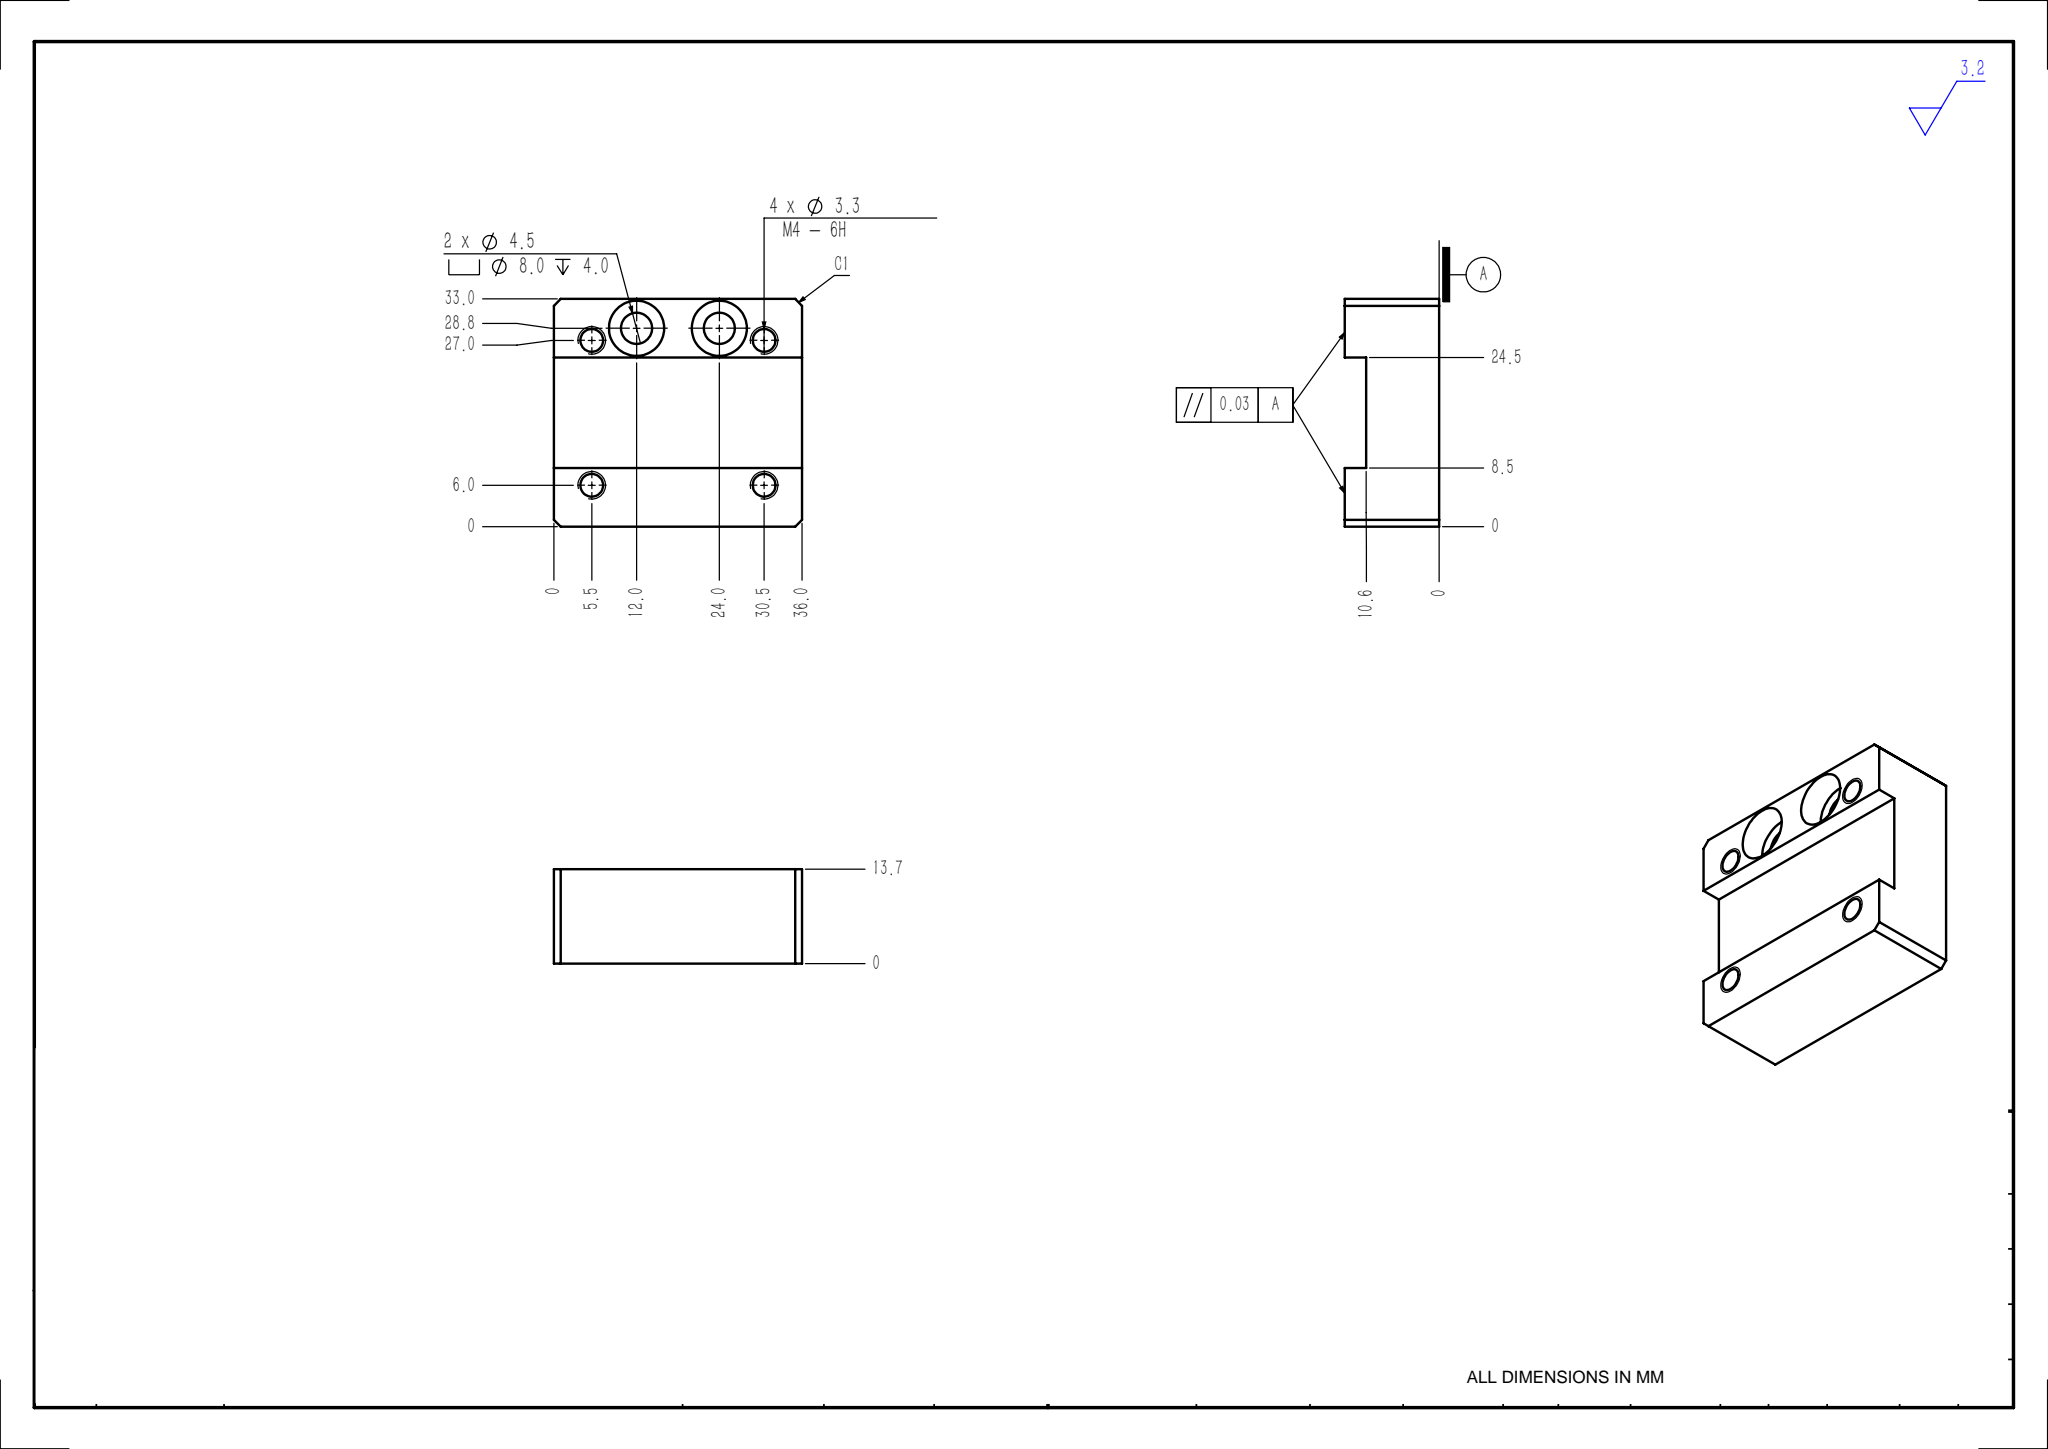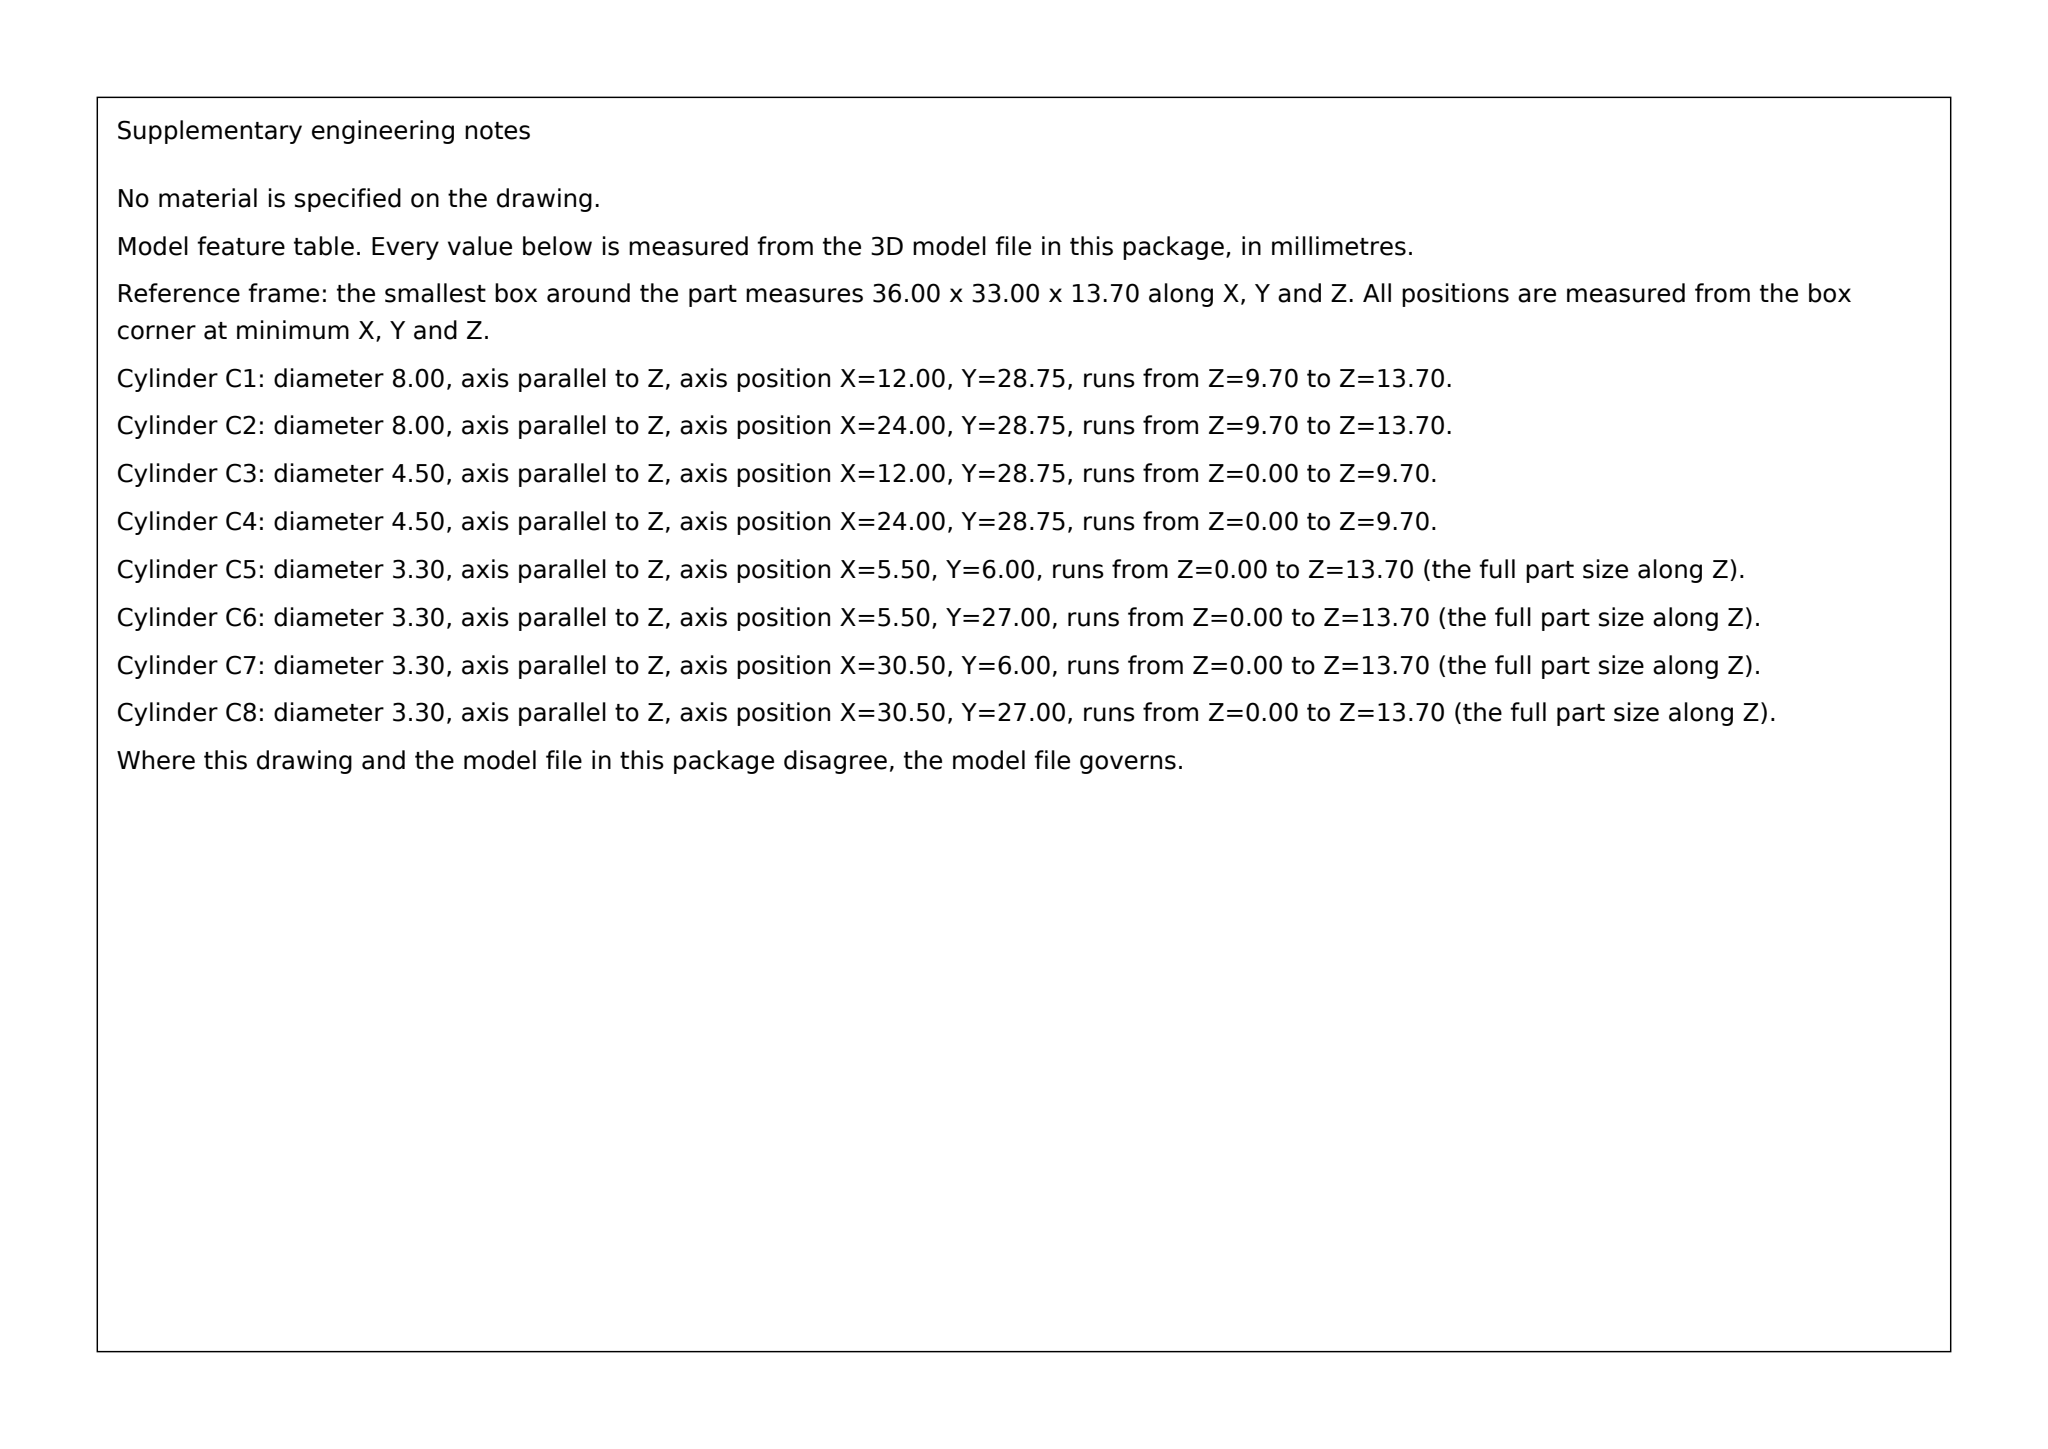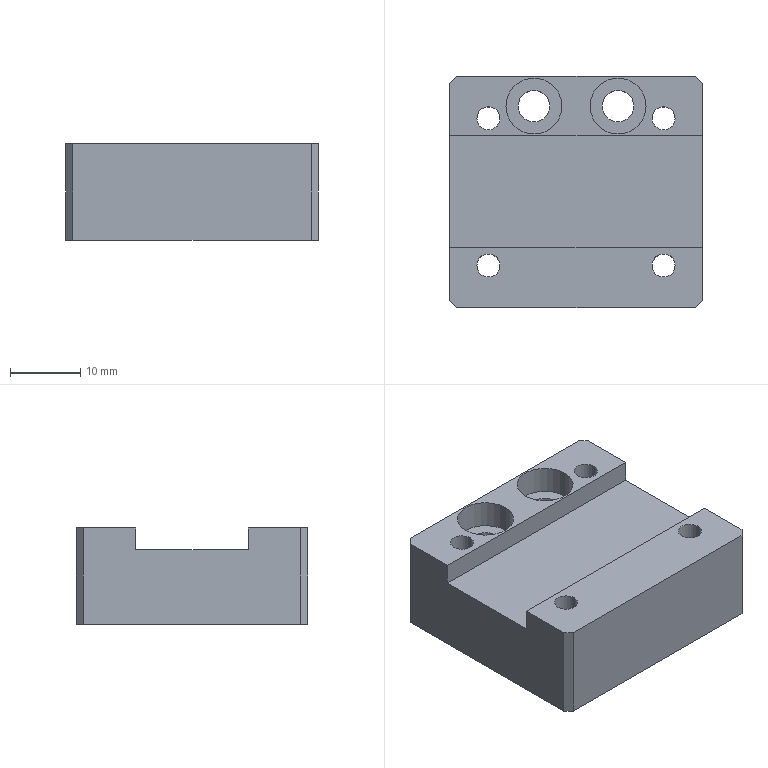Part | SolidWorks | mm | 1 solid | 32 faces | box 36 x 33 x 13.7 mm | volume 13283 mm3 | cylinder 16 | plane 16 | commonest cylinder face diameters 3.3 x8 8 x4 4.5 x4
build123d program:
from build123d import *

# Parameters (mm, degrees)
SKETCH1_W                                            = 36
SKETCH1_H                                            = 33
BOSS_EXTRUDE1_DEPTH                                  = 6.85
SKETCH2_W                                            = 36
SKETCH2_H                                            = 16
CUT_EXTRUDE1_DEPTH                                   = 3.1
M4_TAPPED_HOLE1_D                                    = 3.3
M4_HEX_SOCKET_HEAD_CAP_SCREW_POST_HOLE_2_D           = 4.5
M4_HEX_SOCKET_HEAD_CAP_SCREW_POST_HOLE_2_CBORE_D     = 8
M4_HEX_SOCKET_HEAD_CAP_SCREW_POST_HOLE_2_CBORE_DEPTH = 4
CHAMFER1_SIZE                                        = 1


with BuildPart() as part:
    # Sketch1 → Boss-Extrude1 (new, symmetric)
    with BuildSketch(Plane.XY):
        Rectangle(SKETCH1_W, SKETCH1_H)
    extrude(amount=BOSS_EXTRUDE1_DEPTH, both=True)

    # Sketch2 → Cut-Extrude1 (cut)
    with BuildSketch(Plane.XY.offset(6.85)):
        Rectangle(SKETCH2_W, SKETCH2_H)
    extrude(amount=-CUT_EXTRUDE1_DEPTH, mode=Mode.SUBTRACT)

    # M4 Tapped Hole1 (through all)
    with Locations(Plane.XY.offset(6.85)):
        with Locations((-12.5, 10.5), (12.5, 10.5), (-12.5, -10.5), (12.5, -10.5)):
            Hole(M4_TAPPED_HOLE1_D / 2)

    # M4 Hex Socket Head Cap Screw Post Hole 2 (through all)
    with Locations(Plane.XY.offset(6.85)):
        with Locations((-6, 12.25), (6, 12.25)):
            CounterBoreHole(M4_HEX_SOCKET_HEAD_CAP_SCREW_POST_HOLE_2_D / 2, M4_HEX_SOCKET_HEAD_CAP_SCREW_POST_HOLE_2_CBORE_D / 2, M4_HEX_SOCKET_HEAD_CAP_SCREW_POST_HOLE_2_CBORE_DEPTH)

    # Chamfer1
    chamfer1_edges = [part.edges().sort_by_distance(p)[0] for p in [
        (18, -16.5, 0),
        (-18, -16.5, 0),
        (-18, 16.5, 0),
        (18, 16.5, 0),
    ]]
    chamfer(chamfer1_edges, length=CHAMFER1_SIZE)


solid = part.part